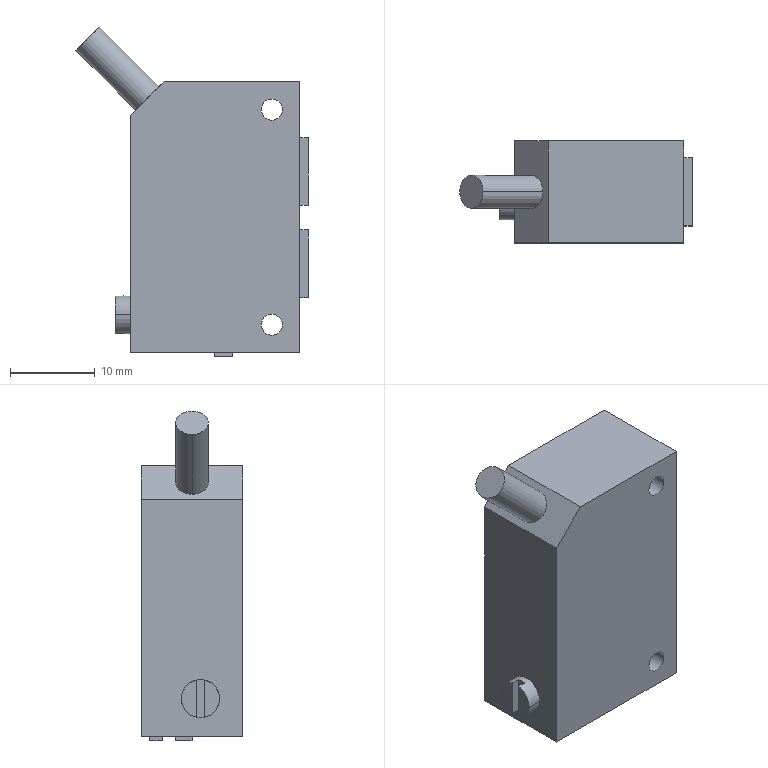Component | SolidWorks | Q20EBanner-2 | 1 solid | 41 faces | box 27.45 x 12 x 38.95 mm | volume 7742 mm3 | plane 33 | cylinder 8 | commonest cylinder face diameters 2.5 x4 4.5 x2 3.9 x2
build123d program:
from build123d import *

# Parameters (mm, degrees)
EXTRUDE1_DEPTH      = 6
EXTRUDE1_DEPTH_BACK = 6
SKETCH1_W           = 20
SKETCH1_H           = 32
M3_TAPPED_HOLE1_D   = 2.5
CHAMFER1_SIZE       = 4
SKETCH4_R           = 1.95
EXTRUDE2_DEPTH      = 10
SKETCH5_R           = 2.25
EXTRUDE3_DEPTH      = 1.8
CUT_EXTRUDE1_START  = -1
CUT_EXTRUDE1_DEPTH  = 1
SKETCH12_W          = 2.2
SKETCH12_H          = 1.5
SKETCH12_H_2        = 1.92
EXTRUDE5_DEPTH      = 0.5
SKETCH9_W           = 8
SKETCH9_H           = 8
EXTRUDE6_DEPTH      = 1


with BuildPart() as part:
    # Sketch1 → Extrude1 (new, two sides: drawn at the far end of the back side and taken through both)
    with BuildSketch(Plane.XY.offset(-EXTRUDE1_DEPTH_BACK)):
        with Locations((10, 16)):
            Rectangle(SKETCH1_W, SKETCH1_H)
    extrude(amount=EXTRUDE1_DEPTH + EXTRUDE1_DEPTH_BACK)

    # M3 Tapped Hole1 (through all)
    with Locations(Plane.XY.offset(6)):
        with Locations((3.3, 28.7), (3.3, 3.3)):
            Hole(M3_TAPPED_HOLE1_D / 2)

    # Chamfer1
    chamfer1_edges = [part.edges().sort_by_distance(p)[0] for p in [
        (20, 0, 0),
    ]]
    chamfer(chamfer1_edges, length=CHAMFER1_SIZE)

    # Sketch4 → Extrude2 (add)
    with BuildSketch(Plane(origin=(8, -8, 0), x_dir=(0, 0, -1), z_dir=(0.7071, -0.7071, 0))):
        with Locations(Location((0, 14.141, 0), (0, 0, 90))):
            Circle(SKETCH4_R)
    extrude(amount=EXTRUDE2_DEPTH)

    # Sketch5 → Extrude3 (add)
    with BuildSketch(Plane(origin=(20, 0, 0), x_dir=(0, 0, -1), z_dir=(1, 0, 0))):
        with Locations((-1, 27.5)):
            Circle(SKETCH5_R)
    extrude(amount=EXTRUDE3_DEPTH)

    # Sketch6 → Cut-Extrude1 (cut)
    with BuildSketch(Plane(origin=(21.8, 0, 0), x_dir=(0, 0, -1), z_dir=(1, 0, 0)).offset(CUT_EXTRUDE1_START)):
        with BuildLine():
            Line((-1.5, 29.694), (-1.5, 25.306))
            ThreePointArc((-1.5, 25.306), (-1, 25.25), (-0.5, 25.306))
            Line((-0.5, 25.306), (-0.5, 29.694))
            ThreePointArc((-0.5, 29.694), (-1, 29.75), (-1.5, 29.694))
        make_face()
    extrude(amount=CUT_EXTRUDE1_DEPTH, mode=Mode.SUBTRACT)

    # Sketch12 → Extrude5 (add)
    with BuildSketch(Plane(origin=(0, 32, 0), x_dir=(1, 0, 0), z_dir=(0, 1, 0))):
        with Locations((9, 4.25)):
            Rectangle(SKETCH12_W, SKETCH12_H)
        with Locations((9, 0.9598)):
            Rectangle(SKETCH12_W, SKETCH12_H_2)
    extrude(amount=EXTRUDE5_DEPTH)

    # Sketch9 → Extrude6 (add)
    with BuildSketch(Plane.ZY):
        with Locations((0, 21.5)):
            Rectangle(SKETCH9_W, SKETCH9_H)
        with Locations((0, 10.6)):
            Rectangle(SKETCH9_W, SKETCH9_H)
    extrude(amount=EXTRUDE6_DEPTH)


solid = part.part

# Placed as in the assembly
solid = solid.moved(Location((-846.908, -99.092, 301.188), (90, 0, -180)))